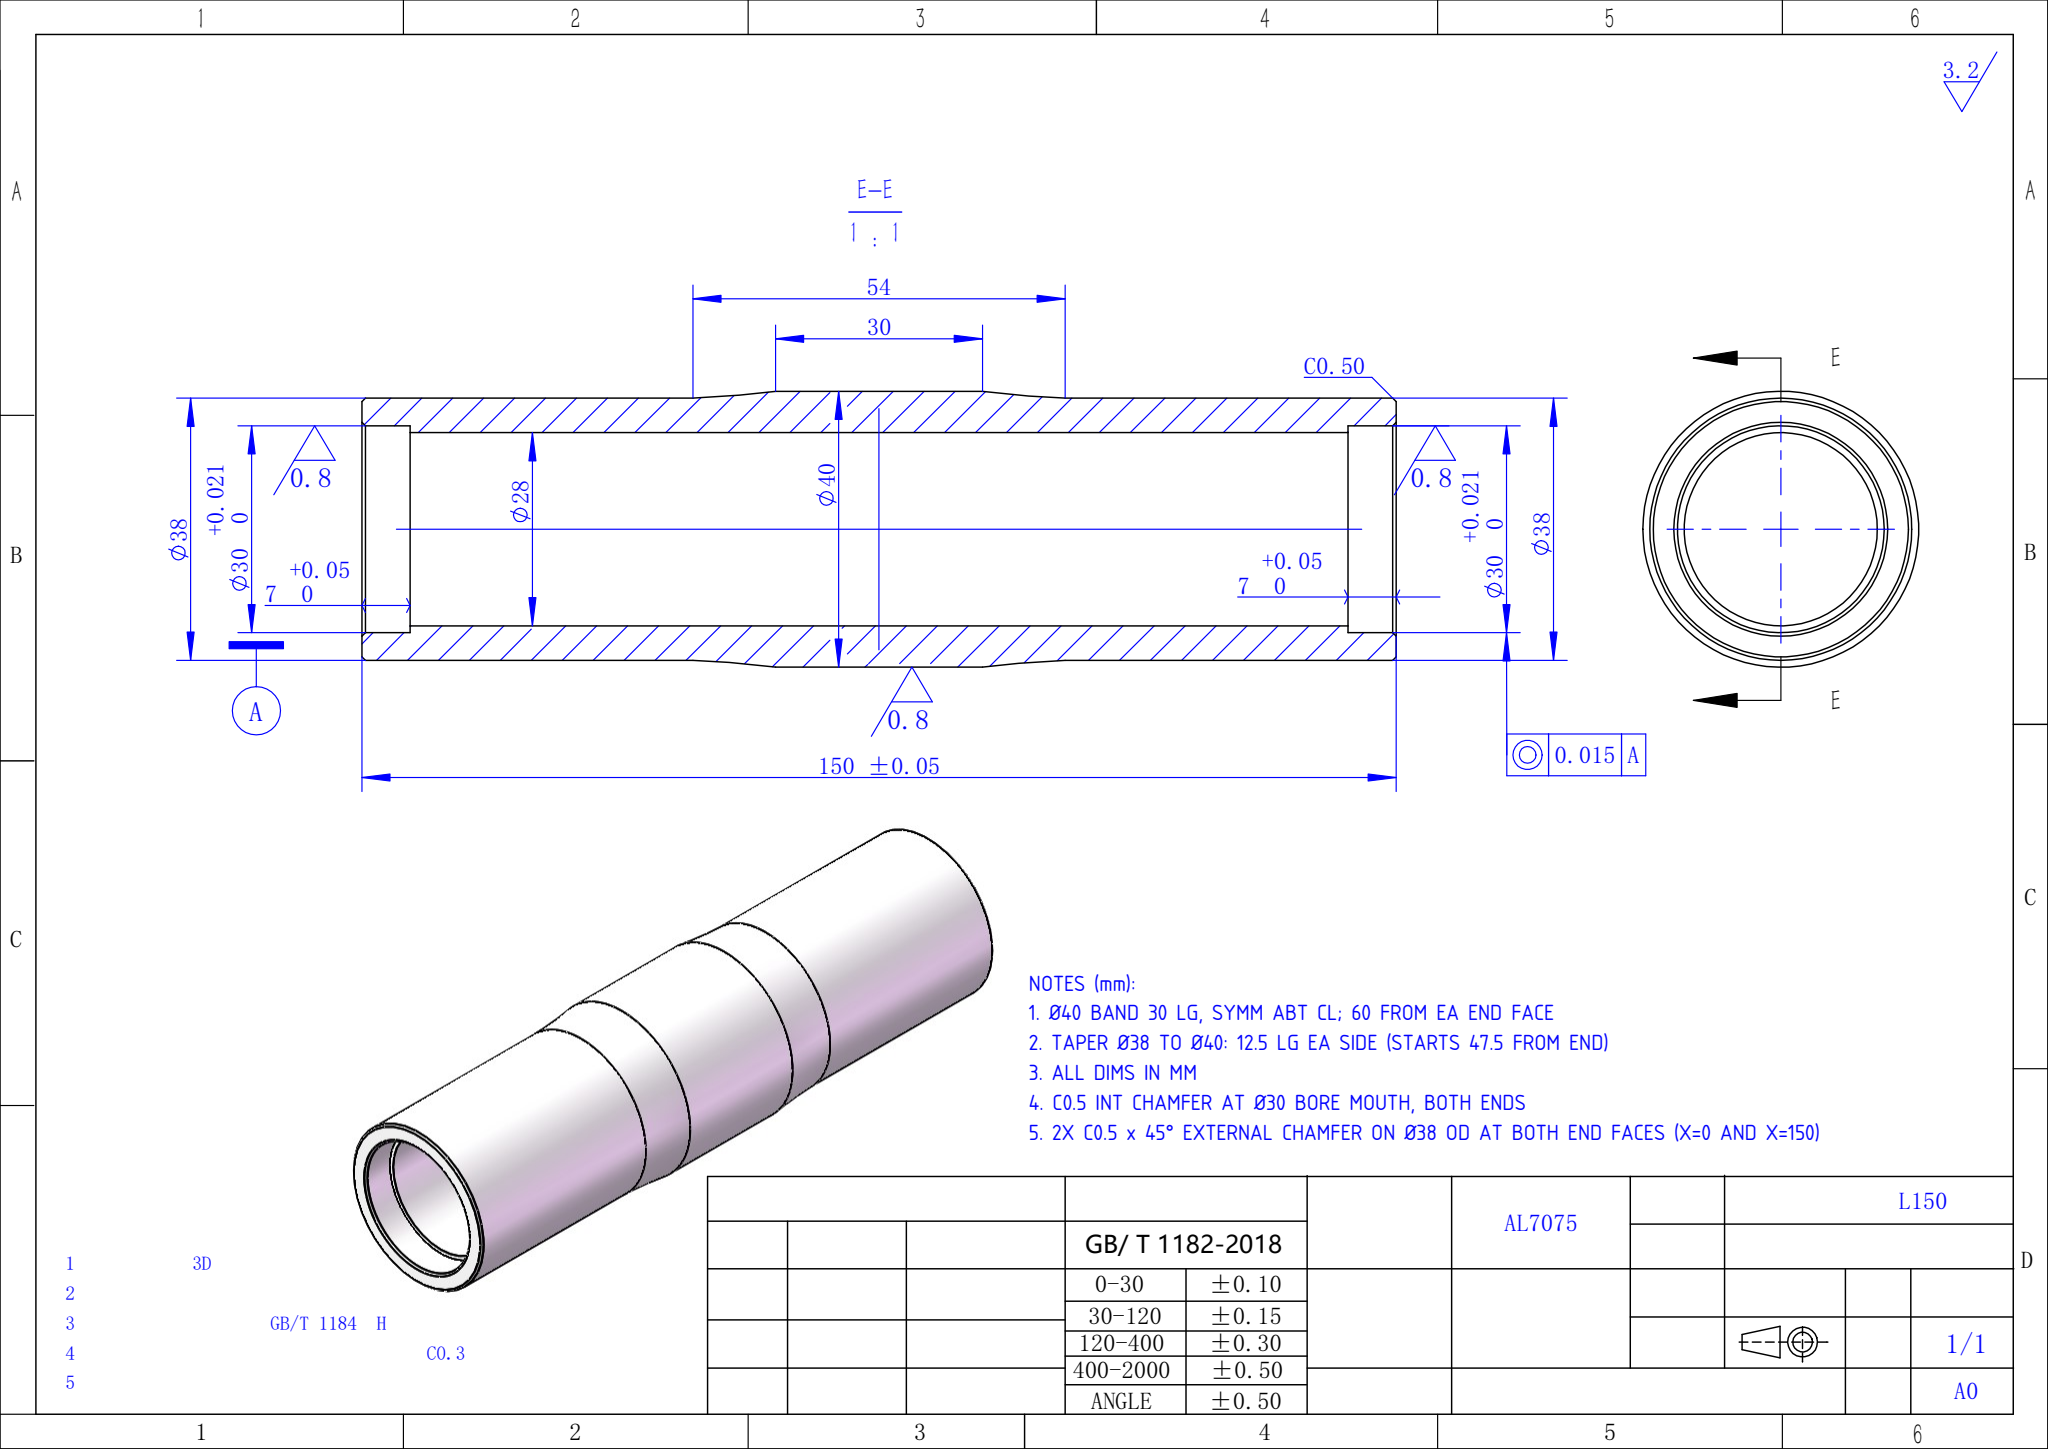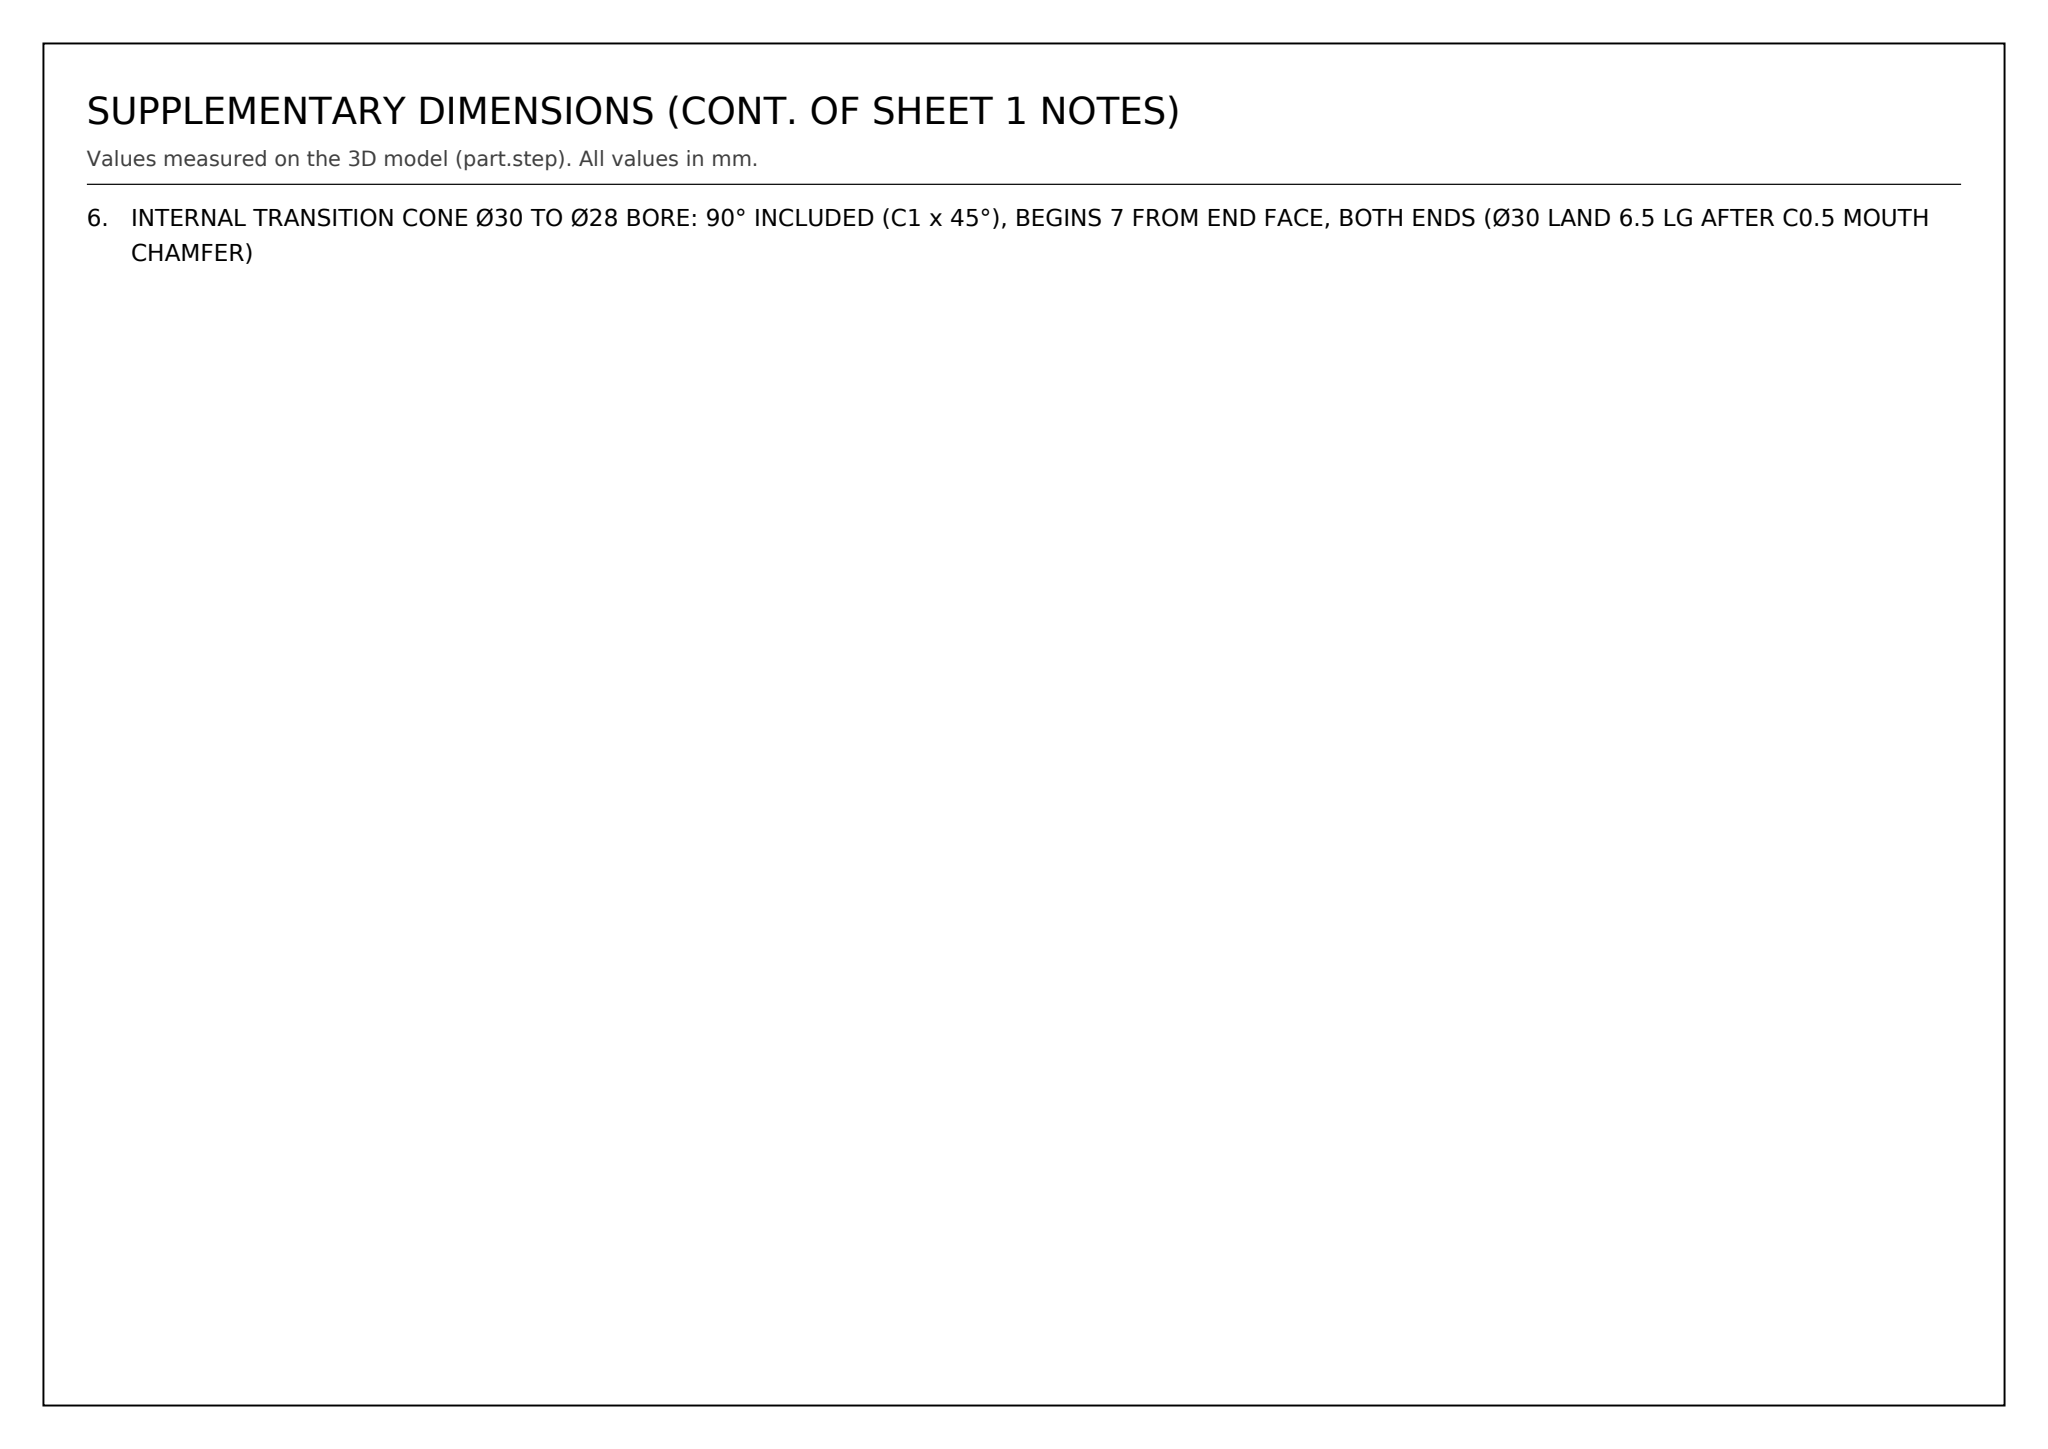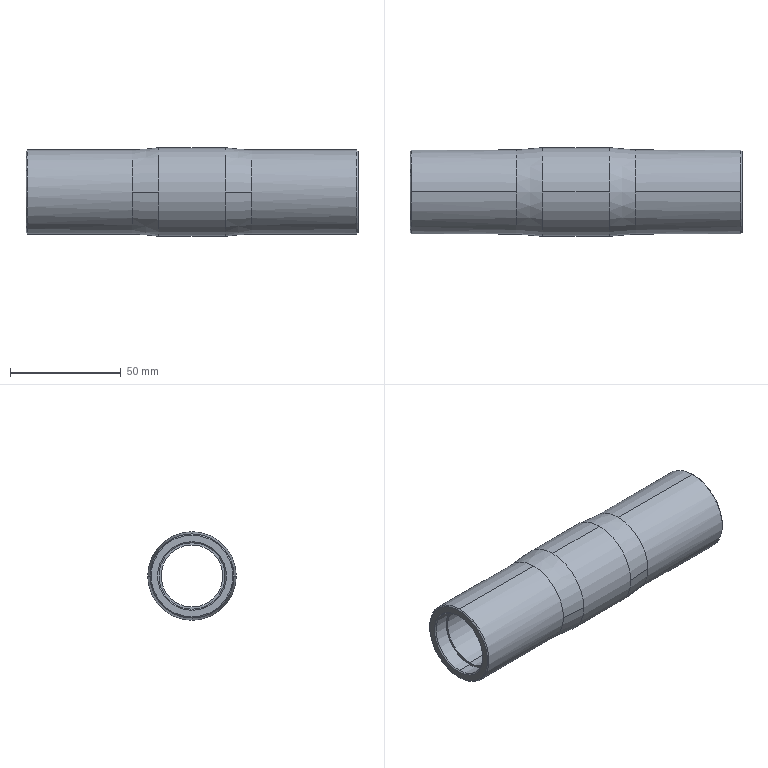Part | SolidWorks | mm | 1 solid | 28 faces | box 150 x 40 x 40 mm | volume 81279 mm3 | cylinder 12 | cone 8 | spline 4 | plane 4 | commonest cylinder face diameters 30 x4 38 x4 40 x2 28 x2
Drawing notes:
Ø40 BAND 30 LG, SYMM ABT CL; 60 FROM EA END FACE | from the solid: Ø40 cyl len 30 on 150 bbox; Ø38 cyl len 47.5 ea end -> band 60 to 90
TAPER Ø38 TO Ø40: 12.5 LG EA SIDE (STARTS 47.5 FROM END) | from the solid: (150-2x47.5-30)/2=12.5 taper len; dia change 38->40
ALL DIMS IN MM | from the solid: STEP model units mm, bbox 150x40x80
C0.5 INT CHAMFER AT Ø30 BORE MOUTH, BOTH ENDS | from the solid: cones 90 deg incl, ref dia 31.0 at Ø30 bore ends (x=0 and x=150), qty 2
2X C0.5 x 45° EXTERNAL CHAMFER ON Ø38 OD AT BOTH END FACES (X=0 AND X=150) | from the solid: cones[90.0 included angle, ref_dia 38.0 -> 37.0], count 2, at axis_planes x=0.0 and x=150.0 bounding the Ø38 cylinders
INTERNAL TRANSITION CONE Ø30 TO Ø28 BORE: 90° INCLUDED (C1 x 45°), BEGINS 7 FROM END FACE, BOTH ENDS (Ø30 LAND 6.5 LG AFTER C0.5 MOUTH CHAMFER) | from the solid: cones[90.0, ref_dia 30.0, count 2]; cylinders Ø30 x-axis length 6.5; axis_planes x=7.0 and x=143.0; Ø28 bore length 136.0
build123d program:
from build123d import *

# Parameters (mm, degrees)
SKETCH2_R          = 14
CUT_EXTRUDE1_DEPTH = 153.643
SKETCH3_R          = 15
CUT_EXTRUDE2_DEPTH = 7
CHAMFER1_SIZE      = 0.5
CHAMFER2_SIZE      = 0.5


with BuildPart() as part:
    # Sketch1 → Revolve1 (revolve)
    with BuildSketch(Plane.XY, mode=Mode.PRIVATE) as revolve1_sk:
        with BuildLine():
            Line((-15, 20), (15, 20))
            add(Edge.make_bspline(
                [(15, 20), (20.992, 19.214), (27, 19)],
                knots=[0, 0, 0, 0.4198, 0.4198, 0.4198], degree=2))
            Line((27, 19), (75, 19))
            Line((75, 19), (75, 0))
            Line((75, 0), (-75, 0))
            Line((-75, 0), (-75, 19))
            Line((-75, 19), (-27, 19))
            add(Edge.make_bspline(
                [(-15, 20), (-20.992, 19.214), (-27, 19)],
                knots=[0, 0, 0, 0.4198, 0.4198, 0.4198], degree=2))
        make_face()
    revolve(revolve1_sk.sketch.rotate(Axis((75, 0, 0), (-1, 0, 0)), 90), axis=Axis((75, 0, 0), (-1, 0, 0)))

    # Sketch2 → Cut-Extrude1 (cut, through all)
    with BuildSketch(Plane(origin=(75, 0, 0), x_dir=(0, 0, -1), z_dir=(1, 0, 0))):
        Circle(SKETCH2_R)
    extrude(amount=-CUT_EXTRUDE1_DEPTH, mode=Mode.SUBTRACT)

    # Sketch3 → Cut-Extrude2 (cut)
    with BuildSketch(Plane(origin=(75, 0, 0), x_dir=(0, 0, -1), z_dir=(1, 0, 0))):
        Circle(SKETCH3_R)
    cut_extrude2 = extrude(amount=-CUT_EXTRUDE2_DEPTH, mode=Mode.SUBTRACT)

    # Chamfer1
    chamfer1_edges = [part.edges().sort_by_distance(p)[0] for p in [
        (75, 0, 15),
        (75, 0, 19),
    ]]
    chamfer(chamfer1_edges, length=CHAMFER1_SIZE)

    # Mirror2: Cut-Extrude2 across plane
    add(cut_extrude2.mirror(Plane(origin=(0, 0, 0), x_dir=(0, 0, 1), z_dir=(1, 0, 0))), mode=Mode.SUBTRACT)

    # Chamfer2
    chamfer2_edges = [part.edges().sort_by_distance(p)[0] for p in [
        (-75, 0, 15),
        (-75, 0, 19),
    ]]
    chamfer(chamfer2_edges, length=CHAMFER2_SIZE)


solid = part.part